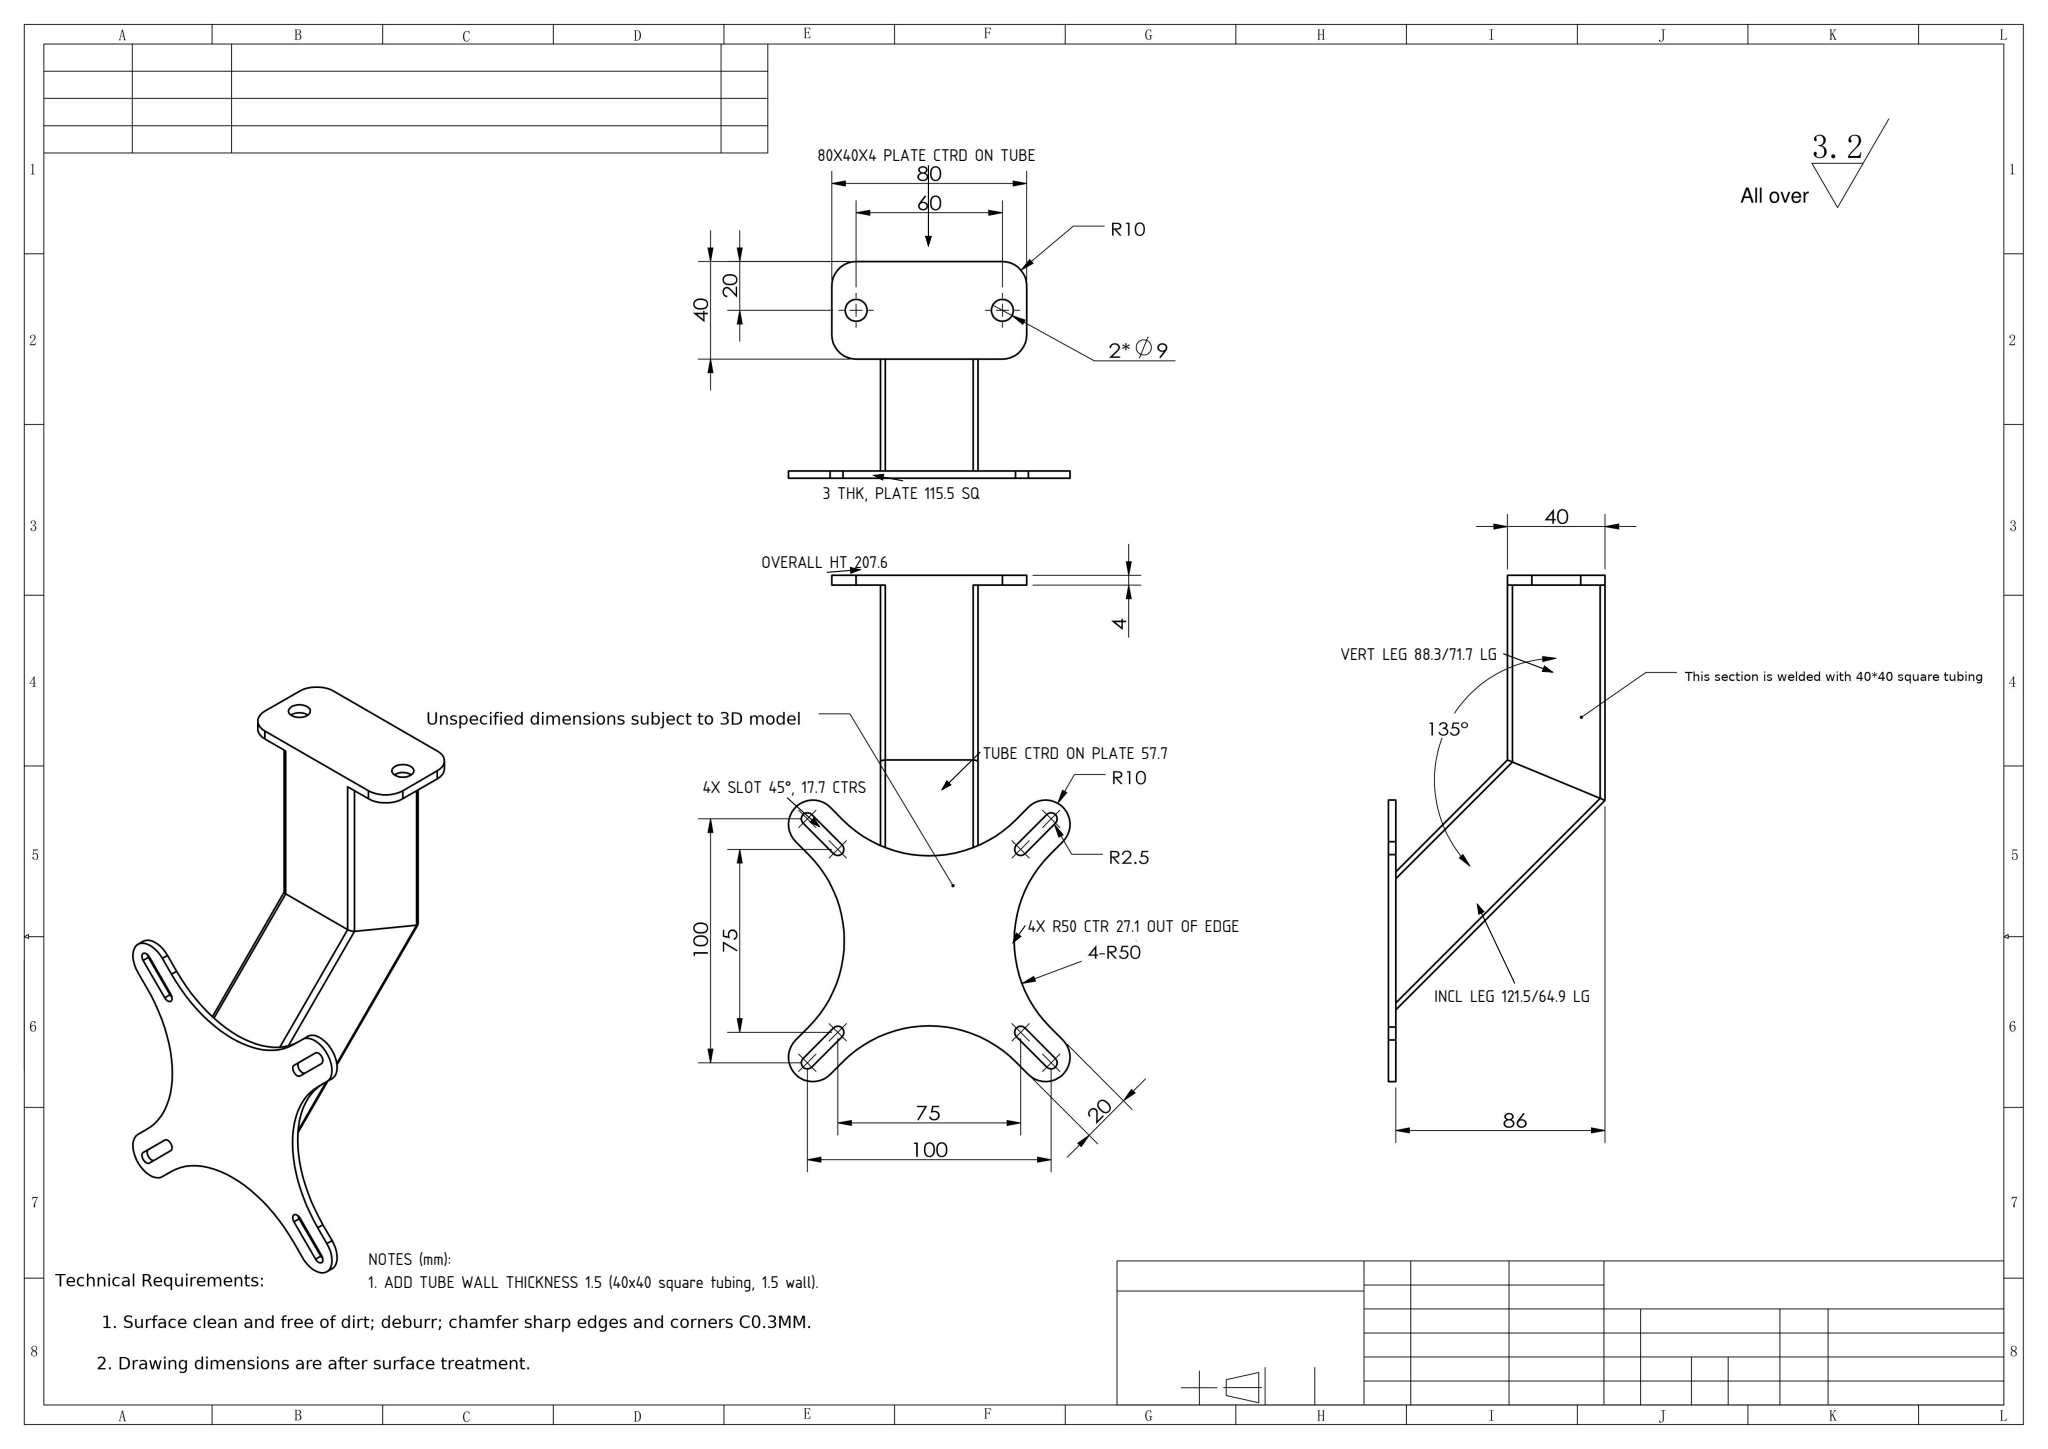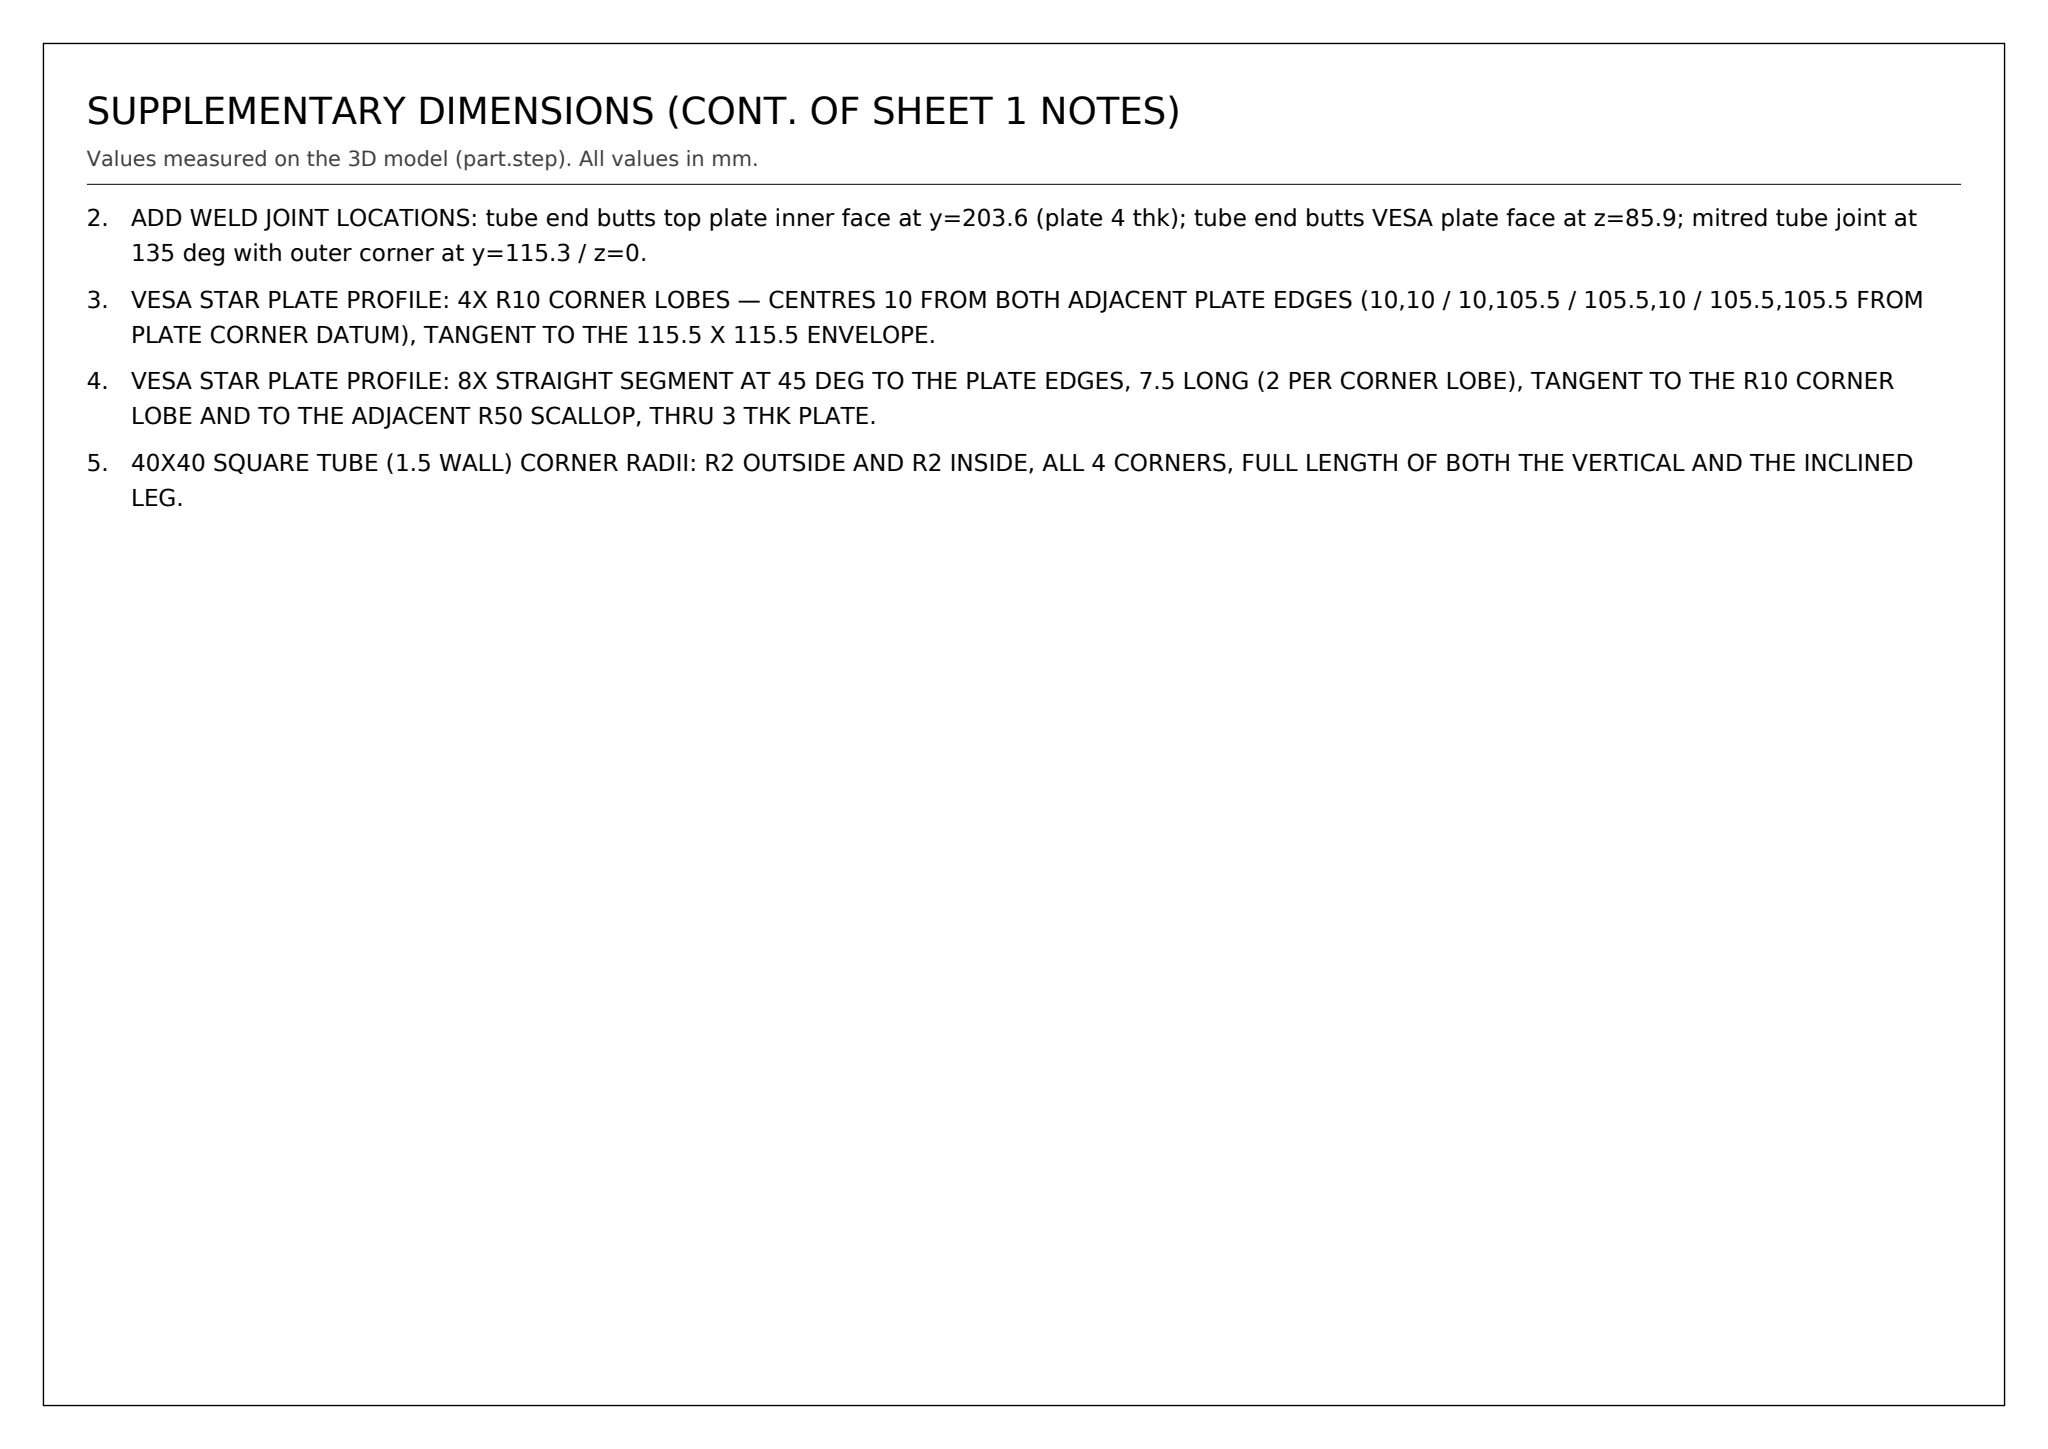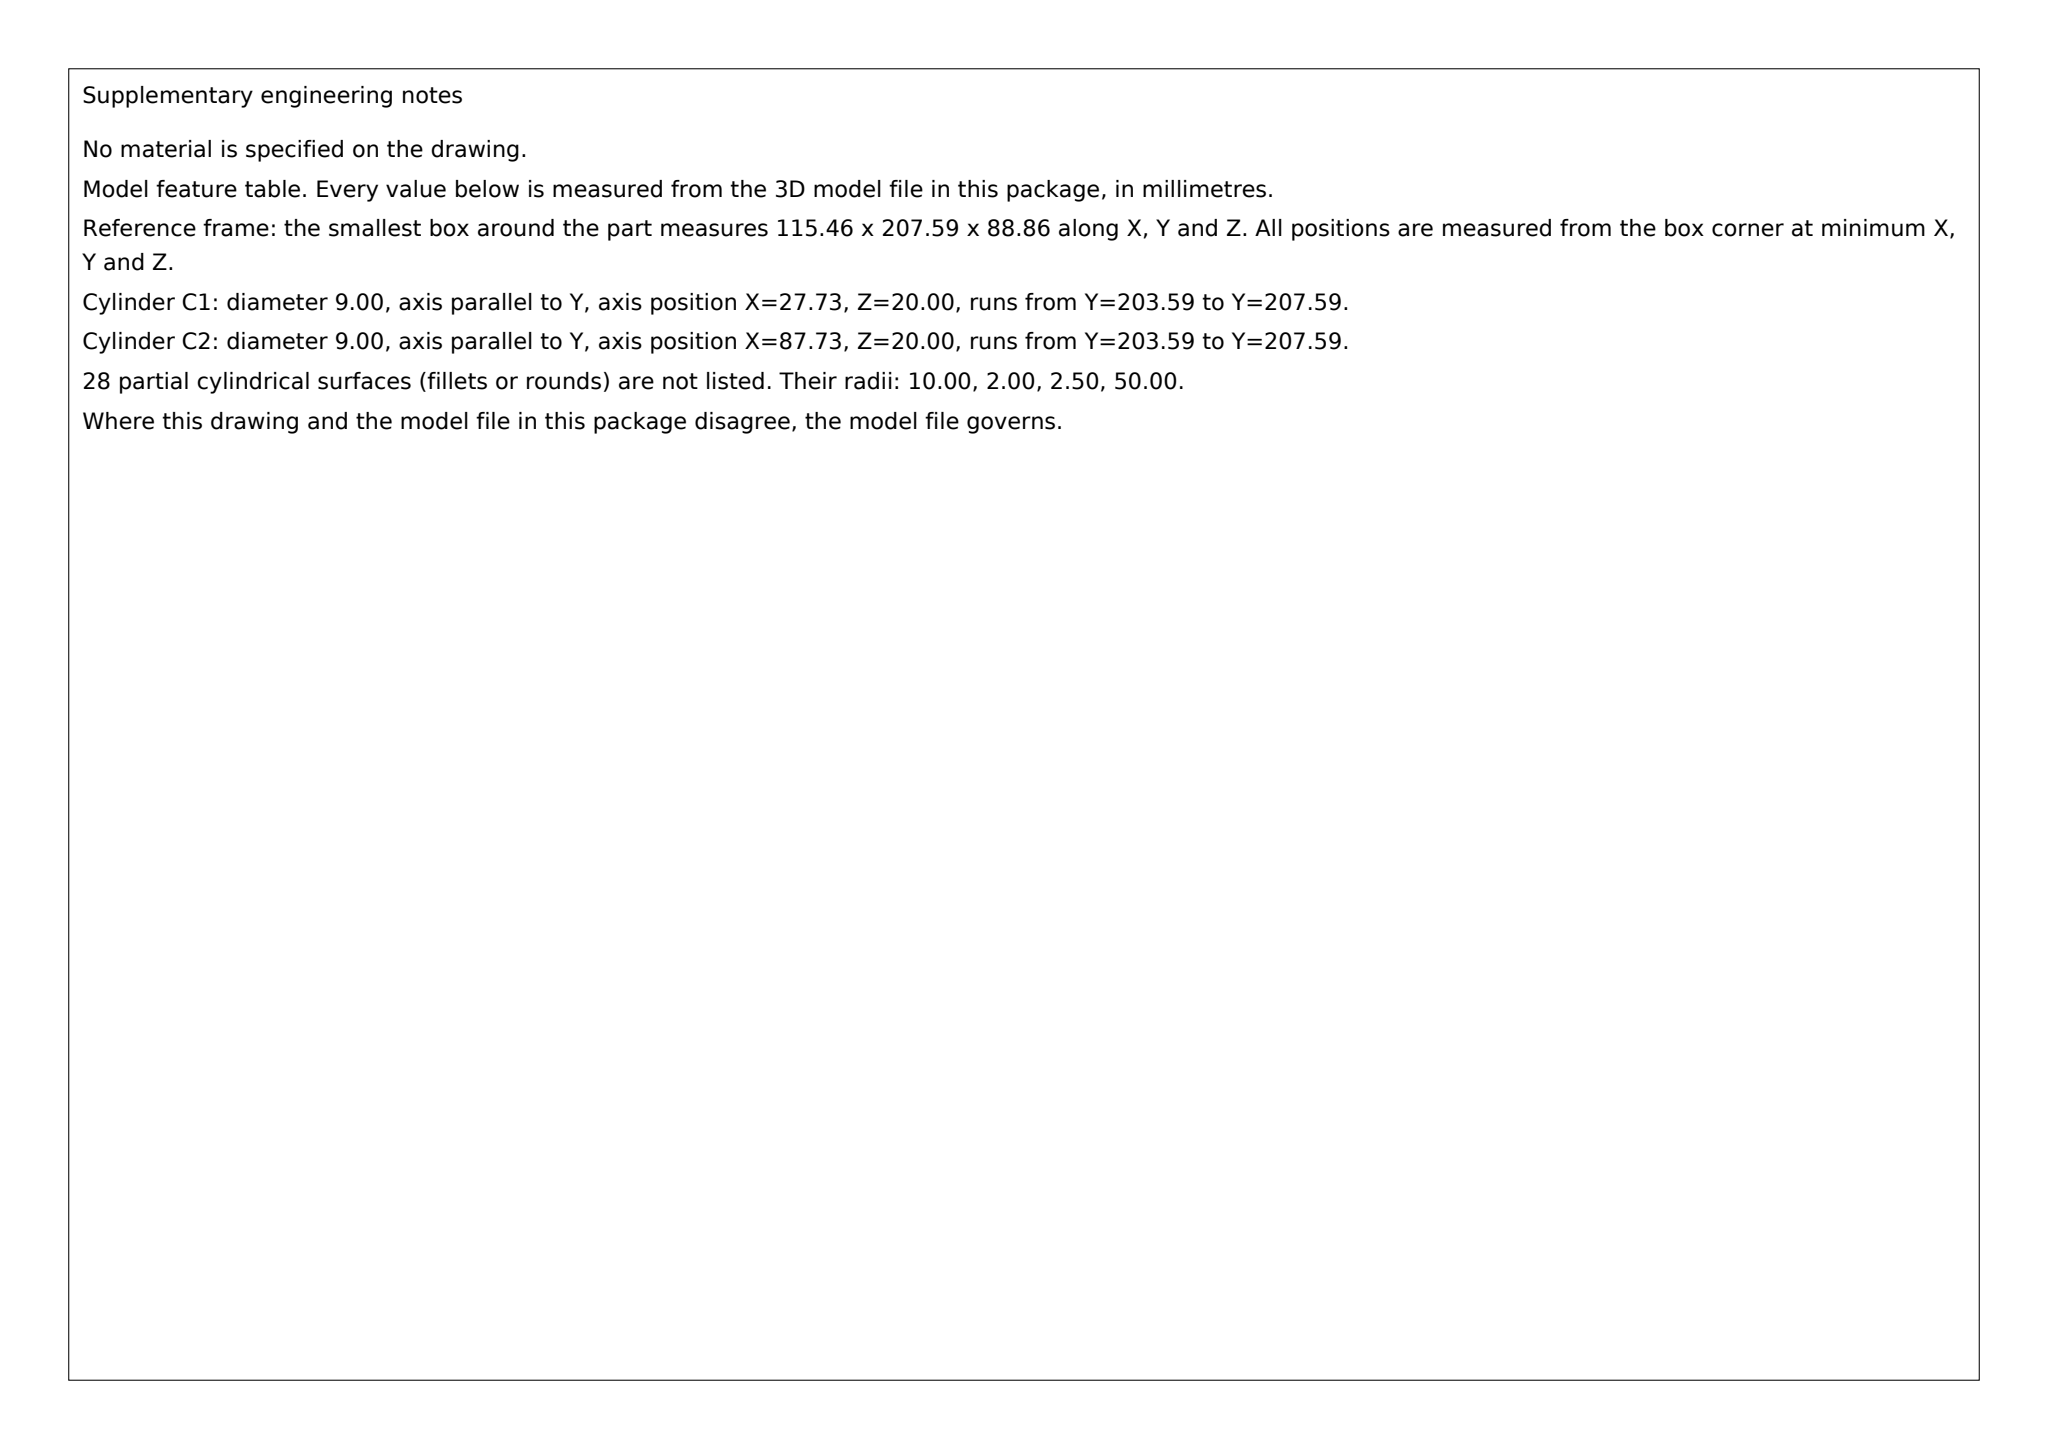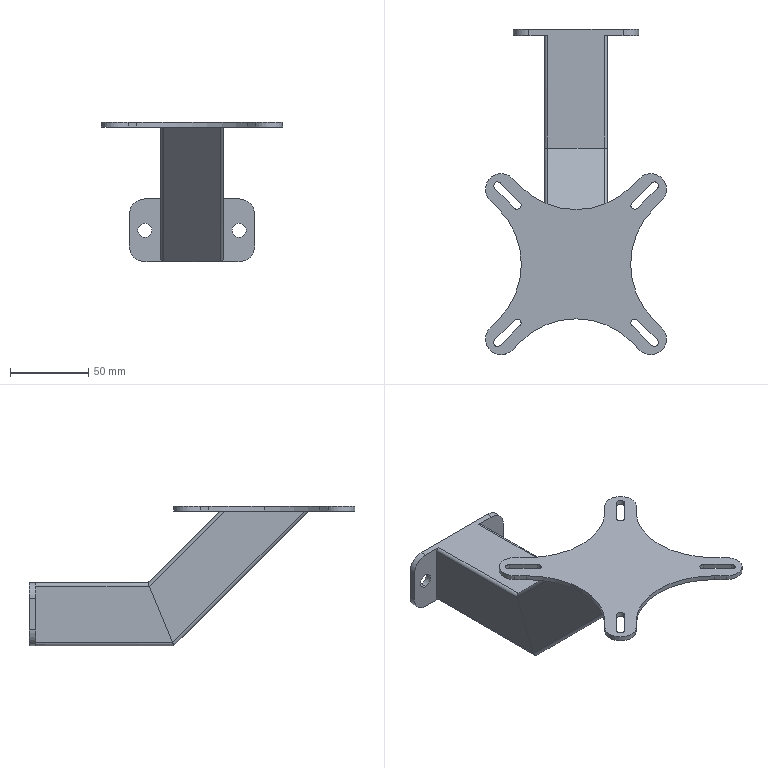Part | SolidWorks | mm | material 40x40x3.5 Square Tube | 1 solid | 88 faces | box 115.46 x 207.59 x 88.86 mm | volume 73969 mm3 | cylinder 47 | plane 41 | commonest cylinder face diameters 4 x16 5 x12 20 x10 100 x5 9 x4
Drawing notes:
ADD OVERALL HEIGHT 207.6 — from outer face of the 80x40 top mounting plate to the far edge of the VESA star plate. | from the solid: bbox_xyz y-extent = 207.588 (top plate outer face y=207.6 to star plate edge y=0)
ADD UPPER (VERTICAL) 40x40 TUBE LEG LENGTH: 88.3 long side / 71.7 short side, measured from the underside of the top plate (y=203.6) to the 135 deg mitre. | from the solid: axis_plane x=37.7 extent y[116.1,203.6] (straight leg side face) and plane z=40 extent y[131.9,207.6]; mitre corners y=115.3 at z=0 and y=131.9 at z=40
ADD INCLINED 40x40 TUBE LEG LENGTH: 121.5 long side / 64.9 short side, from the 135 deg mitre to the face of the VESA star plate (z=85.9). | from the solid: inclined_planes [90,45,45] bbox_from [39.7,29.4,0] size [36,85.9,85.9] and bbox_from [39.7,86.0,40] size [36,45.9,45.9]
ADD TUBE WALL THICKNESS 1.5 (40x40 square tubing, 1.5 wall). | from the solid: axis_planes x=37.7 (outer) vs x=39.2 (inner) and x=77.7 vs x=76.2; z=0 outer vs z=1.5 inner
ADD VESA STAR PLATE THICKNESS 3 (plate 115.5 x 115.5 overall). | from the solid: axis_planes z=85.9 and z=88.9, both extent x[0,115.5] y[0,115.5]
ADD NOTE: 80x40x4 TOP PLATE CENTRED ON TUBE — common centreline x=57.7, 20 overhang each side; plate side faces flush with tube faces (z=0 and z=40). | from the solid: axis_plane y=207.6 extent x[17.7,97.7] z[0,40] (plate) vs tube outer planes x=37.7/77.7, z=0/40
ADD NOTE: TUBE END CENTRED ON VESA PLATE — tube axis meets plate at plate centre x=57.7, y=57.7 from plate corner (tube end spans y 29.4 to 86.0). | from the solid: star plate planes z=85.9/88.9 extent x[0,115.5] y[0,115.5]; inclined tube end faces at y=29.4 and y=86.0, tube x 37.7-77.7
ADD SLOT ORIENTATION: 4 SLOTS AT 45 deg TO THE 100x100 PATTERN (slot axes on the plate diagonals, 17.7 between end-radius centres). | from the solid: slot end cylinders dia 5.0 axis z at (107.7,107.7)/(95.2,95.2), (107.7,7.7)/(95.2,20.2), (20.2,20.2)/(7.7,7.7), (20.2,95.2)/(7.7,107.7) - all pairs on 45 deg lines
ADD WELD JOINT LOCATIONS: tube end butts top plate inner face at y=203.6 (plate 4 thk); tube end butts VESA plate face at z=85.9; mitred tube joint at 135 deg with outer corner at y=115.3 / z=0. | from the solid: axis_planes y=203.6 (plate inner face, tube ends x39.2-76.2 z1.5-38.5) and z=85.9 extent x[39.2,76.2] y[31.6,83.9]; mitre corners y=115.3 (z=0) and y=131.9 (z=40)
VESA STAR PLATE PROFILE: 4X R50 SCALLOPS — ARC CENTRES LIE ON THE PLATE CENTRELINES (X=57.7 AND Y=57.7 FROM PLATE CORNER DATUM) AND 27.1 OUTSIDE THE RESPECTIVE 115.5 PLATE EDGE; SCALLOP APEX THEREFORE 22.9 INBOARD OF THAT EDGE. | from the solid: cylinders: 4X concave arc dia 100.0 (R50), axis z, centres (-27.1,57.7), (142.6,57.7), (57.7,-27.1), (57.7,142.6), from z=85.9 to 88.9; plate face plane z=85.9/88.9 extent x,y 0..115.5
VESA STAR PLATE PROFILE: 4X R10 CORNER LOBES — CENTRES 10 FROM BOTH ADJACENT PLATE EDGES (10,10 / 10,105.5 / 105.5,10 / 105.5,105.5 FROM PLATE CORNER DATUM), TANGENT TO THE 115.5 X 115.5 ENVELOPE. | from the solid: cylinders: 4X convex arc dia 20.0 (R10), axis z, centres (10.0,10.0), (10.0,105.5), (105.5,10.0), (105.5,105.5), from z=85.9 to 88.9, 180 deg
VESA STAR PLATE PROFILE: 8X STRAIGHT SEGMENT AT 45 DEG TO THE PLATE EDGES, 7.5 LONG (2 PER CORNER LOBE), TANGENT TO THE R10 CORNER LOBE AND TO THE ADJACENT R50 SCALLOP, THRU 3 THK PLATE. | from the solid: inclined_planes angle_to_xyz_axes [45,45,90], 8 off, size 5.3 x 5.3 x 3.0, e.g. bbox_from (2.9,17.1,85.9) and (17.1,2.9,85.9) — 5.3*sqrt2 = 7.5 face length, tangent to R10 centre (10,10) and R50 centre (-27.1,57.7)
40X40 SQUARE TUBE (1.5 WALL) CORNER RADII: R2 OUTSIDE AND R2 INSIDE, ALL 4 CORNERS, FULL LENGTH OF BOTH THE VERTICAL AND THE INCLINED LEG. | from the solid: cylinders: convex arc dia 4.0 (R2) at tube outer corners, e.g. axis y at (39.7, z=2.0) and (75.7, z=38.0); concave arc dia 4.0 (R2) at tube inner corners, e.g. axis y at (41.2, z=3.5) and (74.2, z=36.5); tube outer x 37.7-77.7 / z 0-40, inner x 39.2-76.2 / z 1.5-38.5